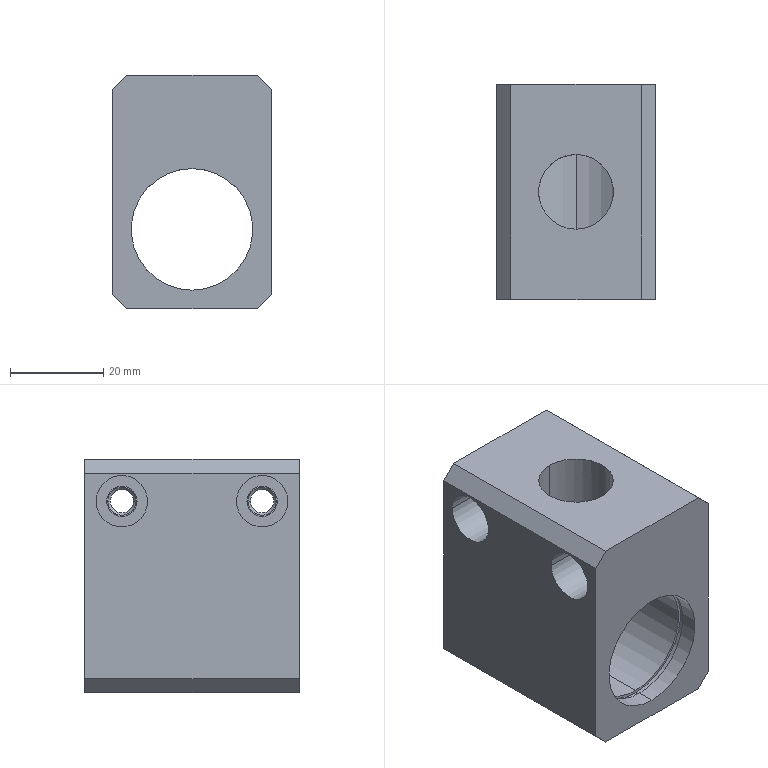Component | SolidWorks | SlidingBearingHousing-2 | 1 solid | 46 faces | box 34 x 46 x 50 mm | volume 45660 mm3 | cylinder 24 | plane 18 | cone 4 | commonest cylinder face diameters 26 x6 27.2 x4 6.5 x4 11 x4 5 x4 16 x2
build123d program:
from build123d import *

# Parameters (mm, degrees)
BOSS_EXTRUDE1_DEPTH             = 46
F_16_0_16_DIAMETER_HOLE1_REACH  = 59.602
F_16_0_16_DIAMETER_HOLE1_BORE_R = 8


with BuildPart() as part:
    # Sketch1 → Boss-Extrude1 (new body)
    with BuildSketch(Plane(origin=(0, 0, -23), x_dir=(-1, 0, 0), z_dir=(0, 0, -1))):
        Polygon((-22, -17), (22, -17), (25, -14), (25, 14), (22, 17), (-22, 17), (-25, 14), (-25, -14), align=None)
    extrude(amount=-BOSS_EXTRUDE1_DEPTH)

    # Sketch2 → Cut-Revolve1 (revolve, cut)
    with BuildSketch(Plane.XY.offset(15), mode=Mode.PRIVATE) as cut_revolve1_sk:
        Polygon((18.5, 17), (16, 17), (16, -17), (21.5, -17), (21.5, -9), (19.25, -9), (19.25, 8), (19.025, 8), (18.5, 8.525), align=None)
    revolve(cut_revolve1_sk.sketch.rotate(Axis((16, 17, 15), (0, -1, 0)), 270), axis=Axis((16, 17, 15), (0, -1, 0)), mode=Mode.SUBTRACT)

    # Sketch3 → Cut-Revolve2 (revolve, cut)
    with BuildSketch(Plane.XY.offset(-15), mode=Mode.PRIVATE) as cut_revolve2_sk:
        Polygon((18.5, 17), (16, 17), (16, -17), (21.5, -17), (21.5, -9), (19.25, -9), (19.25, 8), (19.025, 8), (18.5, 8.525), align=None)
    revolve(cut_revolve2_sk.sketch.rotate(Axis((16, 17, -15), (0, -1, 0)), 270), axis=Axis((16, 17, -15), (0, -1, 0)), mode=Mode.SUBTRACT)

    # Sketch4 → Cut-Revolve3 (revolve, cut)
    with BuildSketch(Plane.XZ, mode=Mode.PRIVATE) as cut_revolve3_sk:
        Polygon((5, 23), (-8, 23), (-8, -23), (5, -23), (5, -19.3), (5.6, -19.3), (5.6, -18), (5, -18), (5, 18), (5.6, 18), (5.6, 19.3), (5, 19.3), align=None)
    revolve(cut_revolve3_sk.sketch.rotate(Axis((-8, 0, 23), (0, 0, -1)), 180), axis=Axis((-8, 0, 23), (0, 0, -1)), mode=Mode.SUBTRACT)

    # 16.0 _16_ Diameter Hole1 bore → 16.0 _16_ Diameter Hole1 (cut, up to next)
    with BuildSketch(Plane(origin=(25, 0, 0), x_dir=(0, 0, -1), z_dir=(1, 0, 0)), mode=Mode.PRIVATE) as f_16_0_16_diameter_hole1_sk1:
        Circle(F_16_0_16_DIAMETER_HOLE1_BORE_R)
    f_16_0_16_diameter_hole1_tool1 = extrude(f_16_0_16_diameter_hole1_sk1.sketch, amount=-F_16_0_16_DIAMETER_HOLE1_REACH, mode=Mode.PRIVATE) & part.part
    add(f_16_0_16_diameter_hole1_tool1.solids().sort_by_distance((25, 0, 0))[0], mode=Mode.SUBTRACT)


solid = part.part

# Placed as in the assembly
solid = solid.moved(Location((-36, 125.451, -230.5), (-90, 0, -90)))